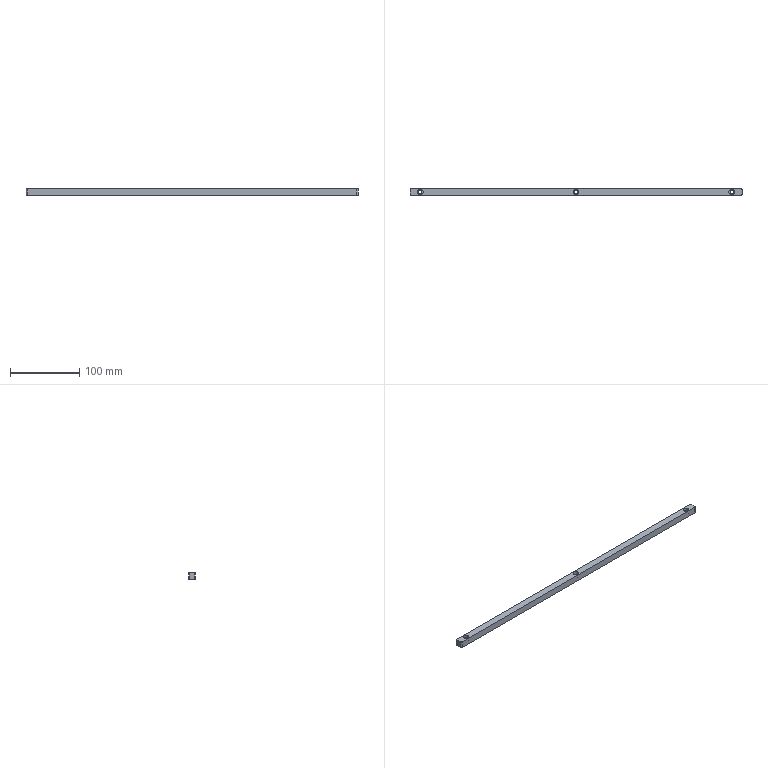Component | SolidWorks | SL010-LeftStreamline-1-1_SL010-02047843SupportBar1-1-1 | 1 solid | 25 faces | box 480 x 10 x 10 mm | volume 47035 mm3 | cylinder 16 | plane 9 | commonest cylinder face diameters 8 x6 4.5 x6 4 x4 | material White POM
STEP:
#1=CARTESIAN_POINT('',(18.937,-4.583,-25.096));
#2=VERTEX_POINT('',#1);
#3=CARTESIAN_POINT('',(19.252,-4.583,-25.096));
#4=VERTEX_POINT('',#3);
#5=CARTESIAN_POINT('',(19.094,-4.583,-25.096));
#6=DIRECTION('',(0.,0.,1.));
#7=DIRECTION('',(1.,0.,0.));
#8=AXIS2_PLACEMENT_3D('',#5,#6,#7);
#9=CIRCLE('',#8,0.1575);
#10=EDGE_CURVE('',#2,#4,#9,.T.);
#11=ORIENTED_EDGE('',*,*,#10,.F.);
#12=CARTESIAN_POINT('',(18.937,-4.583,-24.923));
#13=VERTEX_POINT('',#12);
#14=CARTESIAN_POINT('',(18.937,-4.583,-24.923));
#15=DIRECTION('',(0.,0.,1.));
#16=VECTOR('',#15,39.37);
#17=LINE('',#14,#16);
#18=EDGE_CURVE('',#2,#13,#17,.T.);
#19=ORIENTED_EDGE('',*,*,#18,.T.);
#20=CARTESIAN_POINT('',(19.252,-4.583,-24.923));
#21=VERTEX_POINT('',#20);
#22=CARTESIAN_POINT('',(19.094,-4.583,-24.923));
#23=DIRECTION('',(0.,0.,1.));
#24=DIRECTION('',(1.,0.,0.));
#25=AXIS2_PLACEMENT_3D('',#22,#23,#24);
#26=CIRCLE('',#25,0.1575);
#27=EDGE_CURVE('',#13,#21,#26,.T.);
#28=ORIENTED_EDGE('',*,*,#27,.T.);
#29=CARTESIAN_POINT('',(19.252,-4.583,-24.923));
#30=DIRECTION('',(0.,0.,1.));
#31=VECTOR('',#30,39.37);
#32=LINE('',#29,#31);
#33=EDGE_CURVE('',#4,#21,#32,.T.);
#34=ORIENTED_EDGE('',*,*,#33,.F.);
#35=EDGE_LOOP('',(#11,#19,#28,#34));
#36=FACE_OUTER_BOUND('',#35,.T.);
#37=CARTESIAN_POINT('',(19.094,-4.583,-24.923));
#38=DIRECTION('',(0.,0.,1.));
#39=DIRECTION('',(1.,0.,0.));
#40=AXIS2_PLACEMENT_3D('',#37,#38,#39);
#41=CYLINDRICAL_SURFACE('',#40,0.1575);
#42=ADVANCED_FACE('',(#36),#41,.F.);
#43=CARTESIAN_POINT('',(19.006,-4.583,-25.316));
#44=VERTEX_POINT('',#43);
#45=CARTESIAN_POINT('',(19.183,-4.583,-25.316));
#46=VERTEX_POINT('',#45);
#47=CARTESIAN_POINT('',(19.094,-4.583,-25.316));
#48=DIRECTION('',(0.,0.,1.));
#49=DIRECTION('',(1.,0.,0.));
#50=AXIS2_PLACEMENT_3D('',#47,#48,#49);
#51=CIRCLE('',#50,0.08858);
#52=EDGE_CURVE('',#44,#46,#51,.T.);
#53=ORIENTED_EDGE('',*,*,#52,.F.);
#54=CARTESIAN_POINT('',(19.006,-4.583,-25.096));
#55=VERTEX_POINT('',#54);
#56=CARTESIAN_POINT('',(19.006,-4.583,-24.923));
#57=DIRECTION('',(0.,0.,1.));
#58=VECTOR('',#57,39.37);
#59=LINE('',#56,#58);
#60=EDGE_CURVE('',#44,#55,#59,.T.);
#61=ORIENTED_EDGE('',*,*,#60,.T.);
#62=CARTESIAN_POINT('',(19.183,-4.583,-25.096));
#63=VERTEX_POINT('',#62);
#64=CARTESIAN_POINT('',(19.094,-4.583,-25.096));
#65=DIRECTION('',(0.,0.,1.));
#66=DIRECTION('',(1.,0.,0.));
#67=AXIS2_PLACEMENT_3D('',#64,#65,#66);
#68=CIRCLE('',#67,0.08858);
#69=EDGE_CURVE('',#55,#63,#68,.T.);
#70=ORIENTED_EDGE('',*,*,#69,.T.);
#71=CARTESIAN_POINT('',(19.183,-4.583,-24.923));
#72=DIRECTION('',(0.,0.,1.));
#73=VECTOR('',#72,39.37);
#74=LINE('',#71,#73);
#75=EDGE_CURVE('',#46,#63,#74,.T.);
#76=ORIENTED_EDGE('',*,*,#75,.F.);
#77=EDGE_LOOP('',(#53,#61,#70,#76));
#78=FACE_OUTER_BOUND('',#77,.T.);
#79=CARTESIAN_POINT('',(19.094,-4.583,-24.923));
#80=DIRECTION('',(0.,0.,1.));
#81=DIRECTION('',(1.,0.,0.));
#82=AXIS2_PLACEMENT_3D('',#79,#80,#81);
#83=CYLINDRICAL_SURFACE('',#82,0.08858);
#84=ADVANCED_FACE('',(#78),#83,.F.);
#85=CARTESIAN_POINT('',(36.654,-4.583,-25.096));
#86=VERTEX_POINT('',#85);
#87=CARTESIAN_POINT('',(36.969,-4.583,-25.096));
#88=VERTEX_POINT('',#87);
#89=CARTESIAN_POINT('',(36.811,-4.583,-25.096));
#90=DIRECTION('',(0.,0.,1.));
#91=DIRECTION('',(1.,0.,0.));
#92=AXIS2_PLACEMENT_3D('',#89,#90,#91);
#93=CIRCLE('',#92,0.1575);
#94=EDGE_CURVE('',#86,#88,#93,.T.);
#95=ORIENTED_EDGE('',*,*,#94,.F.);
#96=CARTESIAN_POINT('',(36.654,-4.583,-24.923));
#97=VERTEX_POINT('',#96);
#98=CARTESIAN_POINT('',(36.654,-4.583,-24.923));
#99=DIRECTION('',(0.,0.,1.));
#100=VECTOR('',#99,39.37);
#101=LINE('',#98,#100);
#102=EDGE_CURVE('',#86,#97,#101,.T.);
#103=ORIENTED_EDGE('',*,*,#102,.T.);
#104=CARTESIAN_POINT('',(36.969,-4.583,-24.923));
#105=VERTEX_POINT('',#104);
#106=CARTESIAN_POINT('',(36.811,-4.583,-24.923));
#107=DIRECTION('',(0.,0.,1.));
#108=DIRECTION('',(1.,0.,0.));
#109=AXIS2_PLACEMENT_3D('',#106,#107,#108);
#110=CIRCLE('',#109,0.1575);
#111=EDGE_CURVE('',#97,#105,#110,.T.);
#112=ORIENTED_EDGE('',*,*,#111,.T.);
#113=CARTESIAN_POINT('',(36.969,-4.583,-24.923));
#114=DIRECTION('',(0.,0.,1.));
#115=VECTOR('',#114,39.37);
#116=LINE('',#113,#115);
#117=EDGE_CURVE('',#88,#105,#116,.T.);
#118=ORIENTED_EDGE('',*,*,#117,.F.);
#119=EDGE_LOOP('',(#95,#103,#112,#118));
#120=FACE_OUTER_BOUND('',#119,.T.);
#121=CARTESIAN_POINT('',(36.811,-4.583,-24.923));
#122=DIRECTION('',(0.,0.,1.));
#123=DIRECTION('',(1.,0.,0.));
#124=AXIS2_PLACEMENT_3D('',#121,#122,#123);
#125=CYLINDRICAL_SURFACE('',#124,0.1575);
#126=ADVANCED_FACE('',(#120),#125,.F.);
#127=CARTESIAN_POINT('',(36.722,-4.583,-25.316));
#128=VERTEX_POINT('',#127);
#129=CARTESIAN_POINT('',(36.9,-4.583,-25.316));
#130=VERTEX_POINT('',#129);
#131=CARTESIAN_POINT('',(36.811,-4.583,-25.316));
#132=DIRECTION('',(0.,0.,1.));
#133=DIRECTION('',(1.,0.,0.));
#134=AXIS2_PLACEMENT_3D('',#131,#132,#133);
#135=CIRCLE('',#134,0.08858);
#136=EDGE_CURVE('',#128,#130,#135,.T.);
#137=ORIENTED_EDGE('',*,*,#136,.F.);
#138=CARTESIAN_POINT('',(36.722,-4.583,-25.096));
#139=VERTEX_POINT('',#138);
#140=CARTESIAN_POINT('',(36.722,-4.583,-24.923));
#141=DIRECTION('',(0.,0.,1.));
#142=VECTOR('',#141,39.37);
#143=LINE('',#140,#142);
#144=EDGE_CURVE('',#128,#139,#143,.T.);
#145=ORIENTED_EDGE('',*,*,#144,.T.);
#146=CARTESIAN_POINT('',(36.9,-4.583,-25.096));
#147=VERTEX_POINT('',#146);
#148=CARTESIAN_POINT('',(36.811,-4.583,-25.096));
#149=DIRECTION('',(0.,0.,1.));
#150=DIRECTION('',(1.,0.,0.));
#151=AXIS2_PLACEMENT_3D('',#148,#149,#150);
#152=CIRCLE('',#151,0.08858);
#153=EDGE_CURVE('',#139,#147,#152,.T.);
#154=ORIENTED_EDGE('',*,*,#153,.T.);
#155=CARTESIAN_POINT('',(36.9,-4.583,-24.923));
#156=DIRECTION('',(0.,0.,1.));
#157=VECTOR('',#156,39.37);
#158=LINE('',#155,#157);
#159=EDGE_CURVE('',#130,#147,#158,.T.);
#160=ORIENTED_EDGE('',*,*,#159,.F.);
#161=EDGE_LOOP('',(#137,#145,#154,#160));
#162=FACE_OUTER_BOUND('',#161,.T.);
#163=CARTESIAN_POINT('',(36.811,-4.583,-24.923));
#164=DIRECTION('',(0.,0.,1.));
#165=DIRECTION('',(1.,0.,0.));
#166=AXIS2_PLACEMENT_3D('',#163,#164,#165);
#167=CYLINDRICAL_SURFACE('',#166,0.08858);
#168=ADVANCED_FACE('',(#162),#167,.F.);
#169=CARTESIAN_POINT('',(27.795,-4.583,-25.096));
#170=VERTEX_POINT('',#169);
#171=CARTESIAN_POINT('',(28.11,-4.583,-25.096));
#172=VERTEX_POINT('',#171);
#173=CARTESIAN_POINT('',(27.953,-4.583,-25.096));
#174=DIRECTION('',(0.,0.,1.));
#175=DIRECTION('',(1.,0.,0.));
#176=AXIS2_PLACEMENT_3D('',#173,#174,#175);
#177=CIRCLE('',#176,0.1575);
#178=EDGE_CURVE('',#170,#172,#177,.T.);
#179=ORIENTED_EDGE('',*,*,#178,.F.);
#180=CARTESIAN_POINT('',(27.795,-4.583,-24.923));
#181=VERTEX_POINT('',#180);
#182=CARTESIAN_POINT('',(27.795,-4.583,-24.923));
#183=DIRECTION('',(0.,0.,1.));
#184=VECTOR('',#183,39.37);
#185=LINE('',#182,#184);
#186=EDGE_CURVE('',#170,#181,#185,.T.);
#187=ORIENTED_EDGE('',*,*,#186,.T.);
#188=CARTESIAN_POINT('',(28.11,-4.583,-24.923));
#189=VERTEX_POINT('',#188);
#190=CARTESIAN_POINT('',(27.953,-4.583,-24.923));
#191=DIRECTION('',(0.,0.,1.));
#192=DIRECTION('',(1.,0.,0.));
#193=AXIS2_PLACEMENT_3D('',#190,#191,#192);
#194=CIRCLE('',#193,0.1575);
#195=EDGE_CURVE('',#181,#189,#194,.T.);
#196=ORIENTED_EDGE('',*,*,#195,.T.);
#197=CARTESIAN_POINT('',(28.11,-4.583,-24.923));
#198=DIRECTION('',(0.,0.,1.));
#199=VECTOR('',#198,39.37);
#200=LINE('',#197,#199);
#201=EDGE_CURVE('',#172,#189,#200,.T.);
#202=ORIENTED_EDGE('',*,*,#201,.F.);
#203=EDGE_LOOP('',(#179,#187,#196,#202));
#204=FACE_OUTER_BOUND('',#203,.T.);
#205=CARTESIAN_POINT('',(27.953,-4.583,-24.923));
#206=DIRECTION('',(0.,0.,1.));
#207=DIRECTION('',(1.,0.,0.));
#208=AXIS2_PLACEMENT_3D('',#205,#206,#207);
#209=CYLINDRICAL_SURFACE('',#208,0.1575);
#210=ADVANCED_FACE('',(#204),#209,.F.);
#211=CARTESIAN_POINT('',(27.864,-4.583,-25.316));
#212=VERTEX_POINT('',#211);
#213=CARTESIAN_POINT('',(28.041,-4.583,-25.316));
#214=VERTEX_POINT('',#213);
#215=CARTESIAN_POINT('',(27.953,-4.583,-25.316));
#216=DIRECTION('',(0.,0.,1.));
#217=DIRECTION('',(1.,0.,0.));
#218=AXIS2_PLACEMENT_3D('',#215,#216,#217);
#219=CIRCLE('',#218,0.08858);
#220=EDGE_CURVE('',#212,#214,#219,.T.);
#221=ORIENTED_EDGE('',*,*,#220,.F.);
#222=CARTESIAN_POINT('',(27.864,-4.583,-25.096));
#223=VERTEX_POINT('',#222);
#224=CARTESIAN_POINT('',(27.864,-4.583,-24.923));
#225=DIRECTION('',(0.,0.,1.));
#226=VECTOR('',#225,39.37);
#227=LINE('',#224,#226);
#228=EDGE_CURVE('',#212,#223,#227,.T.);
#229=ORIENTED_EDGE('',*,*,#228,.T.);
#230=CARTESIAN_POINT('',(28.041,-4.583,-25.096));
#231=VERTEX_POINT('',#230);
#232=CARTESIAN_POINT('',(27.953,-4.583,-25.096));
#233=DIRECTION('',(0.,0.,1.));
#234=DIRECTION('',(1.,0.,0.));
#235=AXIS2_PLACEMENT_3D('',#232,#233,#234);
#236=CIRCLE('',#235,0.08858);
#237=EDGE_CURVE('',#223,#231,#236,.T.);
#238=ORIENTED_EDGE('',*,*,#237,.T.);
#239=CARTESIAN_POINT('',(28.041,-4.583,-24.923));
#240=DIRECTION('',(0.,0.,1.));
#241=VECTOR('',#240,39.37);
#242=LINE('',#239,#241);
#243=EDGE_CURVE('',#214,#231,#242,.T.);
#244=ORIENTED_EDGE('',*,*,#243,.F.);
#245=EDGE_LOOP('',(#221,#229,#238,#244));
#246=FACE_OUTER_BOUND('',#245,.T.);
#247=CARTESIAN_POINT('',(27.953,-4.583,-24.923));
#248=DIRECTION('',(0.,0.,1.));
#249=DIRECTION('',(1.,0.,0.));
#250=AXIS2_PLACEMENT_3D('',#247,#248,#249);
#251=CYLINDRICAL_SURFACE('',#250,0.08858);
#252=ADVANCED_FACE('',(#246),#251,.F.);
#253=CARTESIAN_POINT('',(37.402,-4.701,-24.923));
#254=VERTEX_POINT('',#253);
#255=CARTESIAN_POINT('',(37.402,-4.465,-24.923));
#256=VERTEX_POINT('',#255);
#257=CARTESIAN_POINT('',(37.402,-4.386,-24.923));
#258=DIRECTION('',(0.,1.,0.));
#259=VECTOR('',#258,39.37);
#260=LINE('',#257,#259);
#261=EDGE_CURVE('',#254,#256,#260,.T.);
#262=ORIENTED_EDGE('',*,*,#261,.F.);
#263=CARTESIAN_POINT('',(37.402,-4.701,-25.316));
#264=VERTEX_POINT('',#263);
#265=CARTESIAN_POINT('',(37.402,-4.701,-24.923));
#266=DIRECTION('',(0.,0.,-1.));
#267=VECTOR('',#266,39.37);
#268=LINE('',#265,#267);
#269=EDGE_CURVE('',#254,#264,#268,.T.);
#270=ORIENTED_EDGE('',*,*,#269,.T.);
#271=CARTESIAN_POINT('',(37.402,-4.465,-25.316));
#272=VERTEX_POINT('',#271);
#273=CARTESIAN_POINT('',(37.402,-4.386,-25.316));
#274=DIRECTION('',(0.,1.,0.));
#275=VECTOR('',#274,39.37);
#276=LINE('',#273,#275);
#277=EDGE_CURVE('',#264,#272,#276,.T.);
#278=ORIENTED_EDGE('',*,*,#277,.T.);
#279=CARTESIAN_POINT('',(37.402,-4.465,-24.923));
#280=DIRECTION('',(0.,0.,1.));
#281=VECTOR('',#280,39.37);
#282=LINE('',#279,#281);
#283=EDGE_CURVE('',#272,#256,#282,.T.);
#284=ORIENTED_EDGE('',*,*,#283,.T.);
#285=EDGE_LOOP('',(#262,#270,#278,#284));
#286=FACE_OUTER_BOUND('',#285,.T.);
#287=CARTESIAN_POINT('',(37.402,-4.386,-24.923));
#288=DIRECTION('',(-1.,0.,0.));
#289=DIRECTION('',(0.,0.,1.));
#290=AXIS2_PLACEMENT_3D('',#287,#288,#289);
#291=PLANE('',#290);
#292=ADVANCED_FACE('',(#286),#291,.F.);
#293=CARTESIAN_POINT('',(37.323,-4.386,-24.923));
#294=VERTEX_POINT('',#293);
#295=CARTESIAN_POINT('',(18.583,-4.386,-24.923));
#296=VERTEX_POINT('',#295);
#297=CARTESIAN_POINT('',(18.504,-4.386,-24.923));
#298=DIRECTION('',(-1.,0.,0.));
#299=VECTOR('',#298,39.37);
#300=LINE('',#297,#299);
#301=EDGE_CURVE('',#294,#296,#300,.T.);
#302=ORIENTED_EDGE('',*,*,#301,.F.);
#303=CARTESIAN_POINT('',(37.323,-4.386,-25.316));
#304=VERTEX_POINT('',#303);
#305=CARTESIAN_POINT('',(37.323,-4.386,-24.923));
#306=DIRECTION('',(0.,0.,-1.));
#307=VECTOR('',#306,39.37);
#308=LINE('',#305,#307);
#309=EDGE_CURVE('',#294,#304,#308,.T.);
#310=ORIENTED_EDGE('',*,*,#309,.T.);
#311=CARTESIAN_POINT('',(18.583,-4.386,-25.316));
#312=VERTEX_POINT('',#311);
#313=CARTESIAN_POINT('',(18.504,-4.386,-25.316));
#314=DIRECTION('',(-1.,0.,0.));
#315=VECTOR('',#314,39.37);
#316=LINE('',#313,#315);
#317=EDGE_CURVE('',#304,#312,#316,.T.);
#318=ORIENTED_EDGE('',*,*,#317,.T.);
#319=CARTESIAN_POINT('',(18.583,-4.386,-24.923));
#320=DIRECTION('',(0.,0.,1.));
#321=VECTOR('',#320,39.37);
#322=LINE('',#319,#321);
#323=EDGE_CURVE('',#312,#296,#322,.T.);
#324=ORIENTED_EDGE('',*,*,#323,.T.);
#325=EDGE_LOOP('',(#302,#310,#318,#324));
#326=FACE_OUTER_BOUND('',#325,.T.);
#327=CARTESIAN_POINT('',(18.504,-4.386,-24.923));
#328=DIRECTION('',(0.,-1.,0.));
#329=DIRECTION('',(0.,0.,-1.));
#330=AXIS2_PLACEMENT_3D('',#327,#328,#329);
#331=PLANE('',#330);
#332=ADVANCED_FACE('',(#326),#331,.F.);
#333=CARTESIAN_POINT('',(18.504,-4.465,-25.316));
#334=VERTEX_POINT('',#333);
#335=CARTESIAN_POINT('',(18.504,-4.701,-25.316));
#336=VERTEX_POINT('',#335);
#337=CARTESIAN_POINT('',(18.504,-4.386,-25.316));
#338=DIRECTION('',(0.,-1.,0.));
#339=VECTOR('',#338,39.37);
#340=LINE('',#337,#339);
#341=EDGE_CURVE('',#334,#336,#340,.T.);
#342=ORIENTED_EDGE('',*,*,#341,.T.);
#343=CARTESIAN_POINT('',(18.504,-4.701,-24.923));
#344=VERTEX_POINT('',#343);
#345=CARTESIAN_POINT('',(18.504,-4.701,-24.923));
#346=DIRECTION('',(0.,0.,1.));
#347=VECTOR('',#346,39.37);
#348=LINE('',#345,#347);
#349=EDGE_CURVE('',#336,#344,#348,.T.);
#350=ORIENTED_EDGE('',*,*,#349,.T.);
#351=CARTESIAN_POINT('',(18.504,-4.465,-24.923));
#352=VERTEX_POINT('',#351);
#353=CARTESIAN_POINT('',(18.504,-4.386,-24.923));
#354=DIRECTION('',(0.,-1.,0.));
#355=VECTOR('',#354,39.37);
#356=LINE('',#353,#355);
#357=EDGE_CURVE('',#352,#344,#356,.T.);
#358=ORIENTED_EDGE('',*,*,#357,.F.);
#359=CARTESIAN_POINT('',(18.504,-4.465,-24.923));
#360=DIRECTION('',(0.,0.,-1.));
#361=VECTOR('',#360,39.37);
#362=LINE('',#359,#361);
#363=EDGE_CURVE('',#352,#334,#362,.T.);
#364=ORIENTED_EDGE('',*,*,#363,.T.);
#365=EDGE_LOOP('',(#342,#350,#358,#364));
#366=FACE_OUTER_BOUND('',#365,.T.);
#367=CARTESIAN_POINT('',(18.504,-4.386,-24.923));
#368=DIRECTION('',(1.,0.,0.));
#369=DIRECTION('',(0.,0.,-1.));
#370=AXIS2_PLACEMENT_3D('',#367,#368,#369);
#371=PLANE('',#370);
#372=ADVANCED_FACE('',(#366),#371,.F.);
#373=CARTESIAN_POINT('',(18.583,-4.78,-25.316));
#374=VERTEX_POINT('',#373);
#375=CARTESIAN_POINT('',(37.323,-4.78,-25.316));
#376=VERTEX_POINT('',#375);
#377=CARTESIAN_POINT('',(18.504,-4.78,-25.316));
#378=DIRECTION('',(1.,0.,0.));
#379=VECTOR('',#378,39.37);
#380=LINE('',#377,#379);
#381=EDGE_CURVE('',#374,#376,#380,.T.);
#382=ORIENTED_EDGE('',*,*,#381,.T.);
#383=CARTESIAN_POINT('',(37.323,-4.78,-24.923));
#384=VERTEX_POINT('',#383);
#385=CARTESIAN_POINT('',(37.323,-4.78,-24.923));
#386=DIRECTION('',(0.,0.,1.));
#387=VECTOR('',#386,39.37);
#388=LINE('',#385,#387);
#389=EDGE_CURVE('',#376,#384,#388,.T.);
#390=ORIENTED_EDGE('',*,*,#389,.T.);
#391=CARTESIAN_POINT('',(18.583,-4.78,-24.923));
#392=VERTEX_POINT('',#391);
#393=CARTESIAN_POINT('',(18.504,-4.78,-24.923));
#394=DIRECTION('',(1.,0.,0.));
#395=VECTOR('',#394,39.37);
#396=LINE('',#393,#395);
#397=EDGE_CURVE('',#392,#384,#396,.T.);
#398=ORIENTED_EDGE('',*,*,#397,.F.);
#399=CARTESIAN_POINT('',(18.583,-4.78,-24.923));
#400=DIRECTION('',(0.,0.,-1.));
#401=VECTOR('',#400,39.37);
#402=LINE('',#399,#401);
#403=EDGE_CURVE('',#392,#374,#402,.T.);
#404=ORIENTED_EDGE('',*,*,#403,.T.);
#405=EDGE_LOOP('',(#382,#390,#398,#404));
#406=FACE_OUTER_BOUND('',#405,.T.);
#407=CARTESIAN_POINT('',(18.504,-4.78,-24.923));
#408=DIRECTION('',(0.,1.,0.));
#409=DIRECTION('',(0.,0.,1.));
#410=AXIS2_PLACEMENT_3D('',#407,#408,#409);
#411=PLANE('',#410);
#412=ADVANCED_FACE('',(#406),#411,.F.);
#413=CARTESIAN_POINT('',(19.094,-4.583,-24.923));
#414=DIRECTION('',(0.,0.,1.));
#415=DIRECTION('',(1.,0.,0.));
#416=AXIS2_PLACEMENT_3D('',#413,#414,#415);
#417=CIRCLE('',#416,0.1575);
#418=EDGE_CURVE('',#21,#13,#417,.T.);
#419=ORIENTED_EDGE('',*,*,#418,.F.);
#420=ORIENTED_EDGE('',*,*,#27,.F.);
#421=EDGE_LOOP('',(#419,#420));
#422=FACE_BOUND('',#421,.T.);
#423=CARTESIAN_POINT('',(36.811,-4.583,-24.923));
#424=DIRECTION('',(0.,0.,1.));
#425=DIRECTION('',(1.,0.,0.));
#426=AXIS2_PLACEMENT_3D('',#423,#424,#425);
#427=CIRCLE('',#426,0.1575);
#428=EDGE_CURVE('',#105,#97,#427,.T.);
#429=ORIENTED_EDGE('',*,*,#428,.F.);
#430=ORIENTED_EDGE('',*,*,#111,.F.);
#431=EDGE_LOOP('',(#429,#430));
#432=FACE_BOUND('',#431,.T.);
#433=CARTESIAN_POINT('',(27.953,-4.583,-24.923));
#434=DIRECTION('',(0.,0.,1.));
#435=DIRECTION('',(1.,0.,0.));
#436=AXIS2_PLACEMENT_3D('',#433,#434,#435);
#437=CIRCLE('',#436,0.1575);
#438=EDGE_CURVE('',#189,#181,#437,.T.);
#439=ORIENTED_EDGE('',*,*,#438,.F.);
#440=ORIENTED_EDGE('',*,*,#195,.F.);
#441=EDGE_LOOP('',(#439,#440));
#442=FACE_BOUND('',#441,.T.);
#443=ORIENTED_EDGE('',*,*,#397,.T.);
#444=CARTESIAN_POINT('',(37.323,-4.701,-24.923));
#445=DIRECTION('',(0.,0.,1.));
#446=DIRECTION('',(1.,0.,0.));
#447=AXIS2_PLACEMENT_3D('',#444,#445,#446);
#448=CIRCLE('',#447,0.07874);
#449=EDGE_CURVE('',#384,#254,#448,.T.);
#450=ORIENTED_EDGE('',*,*,#449,.T.);
#451=ORIENTED_EDGE('',*,*,#261,.T.);
#452=CARTESIAN_POINT('',(37.323,-4.465,-24.923));
#453=DIRECTION('',(0.,0.,1.));
#454=DIRECTION('',(1.,0.,0.));
#455=AXIS2_PLACEMENT_3D('',#452,#453,#454);
#456=CIRCLE('',#455,0.07874);
#457=EDGE_CURVE('',#256,#294,#456,.T.);
#458=ORIENTED_EDGE('',*,*,#457,.T.);
#459=ORIENTED_EDGE('',*,*,#301,.T.);
#460=CARTESIAN_POINT('',(18.583,-4.465,-24.923));
#461=DIRECTION('',(0.,0.,1.));
#462=DIRECTION('',(1.,0.,0.));
#463=AXIS2_PLACEMENT_3D('',#460,#461,#462);
#464=CIRCLE('',#463,0.07874);
#465=EDGE_CURVE('',#296,#352,#464,.T.);
#466=ORIENTED_EDGE('',*,*,#465,.T.);
#467=ORIENTED_EDGE('',*,*,#357,.T.);
#468=CARTESIAN_POINT('',(18.583,-4.701,-24.923));
#469=DIRECTION('',(0.,0.,1.));
#470=DIRECTION('',(1.,0.,0.));
#471=AXIS2_PLACEMENT_3D('',#468,#469,#470);
#472=CIRCLE('',#471,0.07874);
#473=EDGE_CURVE('',#344,#392,#472,.T.);
#474=ORIENTED_EDGE('',*,*,#473,.T.);
#475=EDGE_LOOP('',(#443,#450,#451,#458,#459,#466,#467,#474));
#476=FACE_OUTER_BOUND('',#475,.T.);
#477=CARTESIAN_POINT('',(27.953,-4.583,-24.923));
#478=DIRECTION('',(0.,0.,1.));
#479=DIRECTION('',(1.,0.,0.));
#480=AXIS2_PLACEMENT_3D('',#477,#478,#479);
#481=PLANE('',#480);
#482=ADVANCED_FACE('',(#422,#432,#442,#476),#481,.T.);
#483=CARTESIAN_POINT('',(19.094,-4.583,-25.316));
#484=DIRECTION('',(0.,0.,1.));
#485=DIRECTION('',(1.,0.,0.));
#486=AXIS2_PLACEMENT_3D('',#483,#484,#485);
#487=CIRCLE('',#486,0.08858);
#488=EDGE_CURVE('',#46,#44,#487,.T.);
#489=ORIENTED_EDGE('',*,*,#488,.T.);
#490=ORIENTED_EDGE('',*,*,#52,.T.);
#491=EDGE_LOOP('',(#489,#490));
#492=FACE_BOUND('',#491,.T.);
#493=CARTESIAN_POINT('',(36.811,-4.583,-25.316));
#494=DIRECTION('',(0.,0.,1.));
#495=DIRECTION('',(1.,0.,0.));
#496=AXIS2_PLACEMENT_3D('',#493,#494,#495);
#497=CIRCLE('',#496,0.08858);
#498=EDGE_CURVE('',#130,#128,#497,.T.);
#499=ORIENTED_EDGE('',*,*,#498,.T.);
#500=ORIENTED_EDGE('',*,*,#136,.T.);
#501=EDGE_LOOP('',(#499,#500));
#502=FACE_BOUND('',#501,.T.);
#503=CARTESIAN_POINT('',(27.953,-4.583,-25.316));
#504=DIRECTION('',(0.,0.,1.));
#505=DIRECTION('',(1.,0.,0.));
#506=AXIS2_PLACEMENT_3D('',#503,#504,#505);
#507=CIRCLE('',#506,0.08858);
#508=EDGE_CURVE('',#214,#212,#507,.T.);
#509=ORIENTED_EDGE('',*,*,#508,.T.);
#510=ORIENTED_EDGE('',*,*,#220,.T.);
#511=EDGE_LOOP('',(#509,#510));
#512=FACE_BOUND('',#511,.T.);
#513=ORIENTED_EDGE('',*,*,#277,.F.);
#514=CARTESIAN_POINT('',(37.323,-4.701,-25.316));
#515=DIRECTION('',(0.,0.,-1.));
#516=DIRECTION('',(1.,0.,0.));
#517=AXIS2_PLACEMENT_3D('',#514,#515,#516);
#518=CIRCLE('',#517,0.07874);
#519=EDGE_CURVE('',#264,#376,#518,.T.);
#520=ORIENTED_EDGE('',*,*,#519,.T.);
#521=ORIENTED_EDGE('',*,*,#381,.F.);
#522=CARTESIAN_POINT('',(18.583,-4.701,-25.316));
#523=DIRECTION('',(0.,0.,-1.));
#524=DIRECTION('',(1.,0.,0.));
#525=AXIS2_PLACEMENT_3D('',#522,#523,#524);
#526=CIRCLE('',#525,0.07874);
#527=EDGE_CURVE('',#374,#336,#526,.T.);
#528=ORIENTED_EDGE('',*,*,#527,.T.);
#529=ORIENTED_EDGE('',*,*,#341,.F.);
#530=CARTESIAN_POINT('',(18.583,-4.465,-25.316));
#531=DIRECTION('',(0.,0.,-1.));
#532=DIRECTION('',(1.,0.,0.));
#533=AXIS2_PLACEMENT_3D('',#530,#531,#532);
#534=CIRCLE('',#533,0.07874);
#535=EDGE_CURVE('',#334,#312,#534,.T.);
#536=ORIENTED_EDGE('',*,*,#535,.T.);
#537=ORIENTED_EDGE('',*,*,#317,.F.);
#538=CARTESIAN_POINT('',(37.323,-4.465,-25.316));
#539=DIRECTION('',(0.,0.,-1.));
#540=DIRECTION('',(1.,0.,0.));
#541=AXIS2_PLACEMENT_3D('',#538,#539,#540);
#542=CIRCLE('',#541,0.07874);
#543=EDGE_CURVE('',#304,#272,#542,.T.);
#544=ORIENTED_EDGE('',*,*,#543,.T.);
#545=EDGE_LOOP('',(#513,#520,#521,#528,#529,#536,#537,#544));
#546=FACE_OUTER_BOUND('',#545,.T.);
#547=CARTESIAN_POINT('',(27.953,-4.583,-25.316));
#548=DIRECTION('',(0.,0.,1.));
#549=DIRECTION('',(1.,0.,0.));
#550=AXIS2_PLACEMENT_3D('',#547,#548,#549);
#551=PLANE('',#550);
#552=ADVANCED_FACE('',(#492,#502,#512,#546),#551,.F.);
#553=ORIENTED_EDGE('',*,*,#228,.F.);
#554=ORIENTED_EDGE('',*,*,#508,.F.);
#555=ORIENTED_EDGE('',*,*,#243,.T.);
#556=CARTESIAN_POINT('',(27.953,-4.583,-25.096));
#557=DIRECTION('',(0.,0.,1.));
#558=DIRECTION('',(1.,0.,0.));
#559=AXIS2_PLACEMENT_3D('',#556,#557,#558);
#560=CIRCLE('',#559,0.08858);
#561=EDGE_CURVE('',#231,#223,#560,.T.);
#562=ORIENTED_EDGE('',*,*,#561,.T.);
#563=EDGE_LOOP('',(#553,#554,#555,#562));
#564=FACE_OUTER_BOUND('',#563,.T.);
#565=CARTESIAN_POINT('',(27.953,-4.583,-24.923));
#566=DIRECTION('',(0.,0.,1.));
#567=DIRECTION('',(1.,0.,0.));
#568=AXIS2_PLACEMENT_3D('',#565,#566,#567);
#569=CYLINDRICAL_SURFACE('',#568,0.08858);
#570=ADVANCED_FACE('',(#564),#569,.F.);
#571=ORIENTED_EDGE('',*,*,#561,.F.);
#572=ORIENTED_EDGE('',*,*,#237,.F.);
#573=EDGE_LOOP('',(#571,#572));
#574=FACE_BOUND('',#573,.T.);
#575=CARTESIAN_POINT('',(27.953,-4.583,-25.096));
#576=DIRECTION('',(0.,0.,1.));
#577=DIRECTION('',(1.,0.,0.));
#578=AXIS2_PLACEMENT_3D('',#575,#576,#577);
#579=CIRCLE('',#578,0.1575);
#580=EDGE_CURVE('',#172,#170,#579,.T.);
#581=ORIENTED_EDGE('',*,*,#580,.T.);
#582=ORIENTED_EDGE('',*,*,#178,.T.);
#583=EDGE_LOOP('',(#581,#582));
#584=FACE_OUTER_BOUND('',#583,.T.);
#585=CARTESIAN_POINT('',(28.041,-4.583,-25.096));
#586=DIRECTION('',(0.,0.,-1.));
#587=DIRECTION('',(-1.,0.,0.));
#588=AXIS2_PLACEMENT_3D('',#585,#586,#587);
#589=PLANE('',#588);
#590=ADVANCED_FACE('',(#574,#584),#589,.F.);
#591=ORIENTED_EDGE('',*,*,#186,.F.);
#592=ORIENTED_EDGE('',*,*,#580,.F.);
#593=ORIENTED_EDGE('',*,*,#201,.T.);
#594=ORIENTED_EDGE('',*,*,#438,.T.);
#595=EDGE_LOOP('',(#591,#592,#593,#594));
#596=FACE_OUTER_BOUND('',#595,.T.);
#597=CARTESIAN_POINT('',(27.953,-4.583,-24.923));
#598=DIRECTION('',(0.,0.,1.));
#599=DIRECTION('',(1.,0.,0.));
#600=AXIS2_PLACEMENT_3D('',#597,#598,#599);
#601=CYLINDRICAL_SURFACE('',#600,0.1575);
#602=ADVANCED_FACE('',(#596),#601,.F.);
#603=ORIENTED_EDGE('',*,*,#144,.F.);
#604=ORIENTED_EDGE('',*,*,#498,.F.);
#605=ORIENTED_EDGE('',*,*,#159,.T.);
#606=CARTESIAN_POINT('',(36.811,-4.583,-25.096));
#607=DIRECTION('',(0.,0.,1.));
#608=DIRECTION('',(1.,0.,0.));
#609=AXIS2_PLACEMENT_3D('',#606,#607,#608);
#610=CIRCLE('',#609,0.08858);
#611=EDGE_CURVE('',#147,#139,#610,.T.);
#612=ORIENTED_EDGE('',*,*,#611,.T.);
#613=EDGE_LOOP('',(#603,#604,#605,#612));
#614=FACE_OUTER_BOUND('',#613,.T.);
#615=CARTESIAN_POINT('',(36.811,-4.583,-24.923));
#616=DIRECTION('',(0.,0.,1.));
#617=DIRECTION('',(1.,0.,0.));
#618=AXIS2_PLACEMENT_3D('',#615,#616,#617);
#619=CYLINDRICAL_SURFACE('',#618,0.08858);
#620=ADVANCED_FACE('',(#614),#619,.F.);
#621=ORIENTED_EDGE('',*,*,#611,.F.);
#622=ORIENTED_EDGE('',*,*,#153,.F.);
#623=EDGE_LOOP('',(#621,#622));
#624=FACE_BOUND('',#623,.T.);
#625=CARTESIAN_POINT('',(36.811,-4.583,-25.096));
#626=DIRECTION('',(0.,0.,1.));
#627=DIRECTION('',(1.,0.,0.));
#628=AXIS2_PLACEMENT_3D('',#625,#626,#627);
#629=CIRCLE('',#628,0.1575);
#630=EDGE_CURVE('',#88,#86,#629,.T.);
#631=ORIENTED_EDGE('',*,*,#630,.T.);
#632=ORIENTED_EDGE('',*,*,#94,.T.);
#633=EDGE_LOOP('',(#631,#632));
#634=FACE_OUTER_BOUND('',#633,.T.);
#635=CARTESIAN_POINT('',(36.9,-4.583,-25.096));
#636=DIRECTION('',(0.,0.,-1.));
#637=DIRECTION('',(-1.,0.,0.));
#638=AXIS2_PLACEMENT_3D('',#635,#636,#637);
#639=PLANE('',#638);
#640=ADVANCED_FACE('',(#624,#634),#639,.F.);
#641=ORIENTED_EDGE('',*,*,#102,.F.);
#642=ORIENTED_EDGE('',*,*,#630,.F.);
#643=ORIENTED_EDGE('',*,*,#117,.T.);
#644=ORIENTED_EDGE('',*,*,#428,.T.);
#645=EDGE_LOOP('',(#641,#642,#643,#644));
#646=FACE_OUTER_BOUND('',#645,.T.);
#647=CARTESIAN_POINT('',(36.811,-4.583,-24.923));
#648=DIRECTION('',(0.,0.,1.));
#649=DIRECTION('',(1.,0.,0.));
#650=AXIS2_PLACEMENT_3D('',#647,#648,#649);
#651=CYLINDRICAL_SURFACE('',#650,0.1575);
#652=ADVANCED_FACE('',(#646),#651,.F.);
#653=ORIENTED_EDGE('',*,*,#60,.F.);
#654=ORIENTED_EDGE('',*,*,#488,.F.);
#655=ORIENTED_EDGE('',*,*,#75,.T.);
#656=CARTESIAN_POINT('',(19.094,-4.583,-25.096));
#657=DIRECTION('',(0.,0.,1.));
#658=DIRECTION('',(1.,0.,0.));
#659=AXIS2_PLACEMENT_3D('',#656,#657,#658);
#660=CIRCLE('',#659,0.08858);
#661=EDGE_CURVE('',#63,#55,#660,.T.);
#662=ORIENTED_EDGE('',*,*,#661,.T.);
#663=EDGE_LOOP('',(#653,#654,#655,#662));
#664=FACE_OUTER_BOUND('',#663,.T.);
#665=CARTESIAN_POINT('',(19.094,-4.583,-24.923));
#666=DIRECTION('',(0.,0.,1.));
#667=DIRECTION('',(1.,0.,0.));
#668=AXIS2_PLACEMENT_3D('',#665,#666,#667);
#669=CYLINDRICAL_SURFACE('',#668,0.08858);
#670=ADVANCED_FACE('',(#664),#669,.F.);
#671=ORIENTED_EDGE('',*,*,#661,.F.);
#672=ORIENTED_EDGE('',*,*,#69,.F.);
#673=EDGE_LOOP('',(#671,#672));
#674=FACE_BOUND('',#673,.T.);
#675=CARTESIAN_POINT('',(19.094,-4.583,-25.096));
#676=DIRECTION('',(0.,0.,1.));
#677=DIRECTION('',(1.,0.,0.));
#678=AXIS2_PLACEMENT_3D('',#675,#676,#677);
#679=CIRCLE('',#678,0.1575);
#680=EDGE_CURVE('',#4,#2,#679,.T.);
#681=ORIENTED_EDGE('',*,*,#680,.T.);
#682=ORIENTED_EDGE('',*,*,#10,.T.);
#683=EDGE_LOOP('',(#681,#682));
#684=FACE_OUTER_BOUND('',#683,.T.);
#685=CARTESIAN_POINT('',(19.183,-4.583,-25.096));
#686=DIRECTION('',(0.,0.,-1.));
#687=DIRECTION('',(-1.,0.,0.));
#688=AXIS2_PLACEMENT_3D('',#685,#686,#687);
#689=PLANE('',#688);
#690=ADVANCED_FACE('',(#674,#684),#689,.F.);
#691=ORIENTED_EDGE('',*,*,#18,.F.);
#692=ORIENTED_EDGE('',*,*,#680,.F.);
#693=ORIENTED_EDGE('',*,*,#33,.T.);
#694=ORIENTED_EDGE('',*,*,#418,.T.);
#695=EDGE_LOOP('',(#691,#692,#693,#694));
#696=FACE_OUTER_BOUND('',#695,.T.);
#697=CARTESIAN_POINT('',(19.094,-4.583,-24.923));
#698=DIRECTION('',(0.,0.,1.));
#699=DIRECTION('',(1.,0.,0.));
#700=AXIS2_PLACEMENT_3D('',#697,#698,#699);
#701=CYLINDRICAL_SURFACE('',#700,0.1575);
#702=ADVANCED_FACE('',(#696),#701,.F.);
#703=ORIENTED_EDGE('',*,*,#449,.F.);
#704=ORIENTED_EDGE('',*,*,#389,.F.);
#705=ORIENTED_EDGE('',*,*,#519,.F.);
#706=ORIENTED_EDGE('',*,*,#269,.F.);
#707=EDGE_LOOP('',(#703,#704,#705,#706));
#708=FACE_OUTER_BOUND('',#707,.T.);
#709=CARTESIAN_POINT('',(37.323,-4.701,-24.923));
#710=DIRECTION('',(0.,0.,-1.));
#711=DIRECTION('',(-1.,0.,0.));
#712=AXIS2_PLACEMENT_3D('',#709,#710,#711);
#713=CYLINDRICAL_SURFACE('',#712,0.07874);
#714=ADVANCED_FACE('',(#708),#713,.T.);
#715=ORIENTED_EDGE('',*,*,#457,.F.);
#716=ORIENTED_EDGE('',*,*,#283,.F.);
#717=ORIENTED_EDGE('',*,*,#543,.F.);
#718=ORIENTED_EDGE('',*,*,#309,.F.);
#719=EDGE_LOOP('',(#715,#716,#717,#718));
#720=FACE_OUTER_BOUND('',#719,.T.);
#721=CARTESIAN_POINT('',(37.323,-4.465,-24.923));
#722=DIRECTION('',(0.,0.,-1.));
#723=DIRECTION('',(-1.,0.,0.));
#724=AXIS2_PLACEMENT_3D('',#721,#722,#723);
#725=CYLINDRICAL_SURFACE('',#724,0.07874);
#726=ADVANCED_FACE('',(#720),#725,.T.);
#727=ORIENTED_EDGE('',*,*,#473,.F.);
#728=ORIENTED_EDGE('',*,*,#349,.F.);
#729=ORIENTED_EDGE('',*,*,#527,.F.);
#730=ORIENTED_EDGE('',*,*,#403,.F.);
#731=EDGE_LOOP('',(#727,#728,#729,#730));
#732=FACE_OUTER_BOUND('',#731,.T.);
#733=CARTESIAN_POINT('',(18.583,-4.701,-24.923));
#734=DIRECTION('',(0.,0.,-1.));
#735=DIRECTION('',(-1.,0.,0.));
#736=AXIS2_PLACEMENT_3D('',#733,#734,#735);
#737=CYLINDRICAL_SURFACE('',#736,0.07874);
#738=ADVANCED_FACE('',(#732),#737,.T.);
#739=ORIENTED_EDGE('',*,*,#465,.F.);
#740=ORIENTED_EDGE('',*,*,#323,.F.);
#741=ORIENTED_EDGE('',*,*,#535,.F.);
#742=ORIENTED_EDGE('',*,*,#363,.F.);
#743=EDGE_LOOP('',(#739,#740,#741,#742));
#744=FACE_OUTER_BOUND('',#743,.T.);
#745=CARTESIAN_POINT('',(18.583,-4.465,-24.923));
#746=DIRECTION('',(0.,0.,-1.));
#747=DIRECTION('',(-1.,0.,0.));
#748=AXIS2_PLACEMENT_3D('',#745,#746,#747);
#749=CYLINDRICAL_SURFACE('',#748,0.07874);
#750=ADVANCED_FACE('',(#744),#749,.T.);
#751=CLOSED_SHELL('',(#42,#84,#126,#168,#210,#252,#292,#332,#372,#412,#482,#552,#570,#590,#602,#620,#640,#652,#670,#690,#702,#714,#726,#738,#750));
#752=MANIFOLD_SOLID_BREP('',#751);
#753=CARTESIAN_POINT('',(0.,0.,0.));
#754=DIRECTION('',(0.,0.,1.));
#755=DIRECTION('',(1.,0.,0.));
#756=AXIS2_PLACEMENT_3D('',#753,#754,#755);
#757=(LENGTH_UNIT()NAMED_UNIT(*)SI_UNIT($,.METRE.));
#758=LENGTH_MEASURE_WITH_UNIT(LENGTH_MEASURE(0.0254),#757);
#759=DIMENSIONAL_EXPONENTS(1.,0.,0.,0.,0.,0.,0.);
#760=(CONVERSION_BASED_UNIT('',#758)LENGTH_UNIT()NAMED_UNIT(#759));
#761=UNCERTAINTY_MEASURE_WITH_UNIT(LENGTH_MEASURE(0.00001),#760,'','');
#762=(NAMED_UNIT(*)PLANE_ANGLE_UNIT()SI_UNIT($,.RADIAN.));
#763=(NAMED_UNIT(*)SI_UNIT($,.STERADIAN.)SOLID_ANGLE_UNIT());
#764=(GEOMETRIC_REPRESENTATION_CONTEXT(3)GLOBAL_UNCERTAINTY_ASSIGNED_CONTEXT((#761))GLOBAL_UNIT_ASSIGNED_CONTEXT((#760,#762,#763))REPRESENTATION_CONTEXT('',''));
#765=ADVANCED_BREP_SHAPE_REPRESENTATION('',(#752,#756),#764);
#766=COLOUR_RGB('',0.7922,0.8196,0.9333);
#767=FILL_AREA_STYLE_COLOUR('',#766);
#768=FILL_AREA_STYLE('',(#767));
#769=SURFACE_STYLE_FILL_AREA(#768);
#770=SURFACE_SIDE_STYLE('',(#769));
#771=SURFACE_STYLE_USAGE(.BOTH.,#770);
#772=PRESENTATION_STYLE_ASSIGNMENT((#771));
#773=STYLED_ITEM('',(#772),#752);
#774=PRESENTATION_LAYER_ASSIGNMENT('','',(#773));
#775=(LENGTH_UNIT()NAMED_UNIT(*)SI_UNIT($,.METRE.));
#776=LENGTH_MEASURE_WITH_UNIT(LENGTH_MEASURE(0.0254),#775);
#777=DIMENSIONAL_EXPONENTS(1.,0.,0.,0.,0.,0.,0.);
#778=(CONVERSION_BASED_UNIT('',#776)LENGTH_UNIT()NAMED_UNIT(#777));
#779=UNCERTAINTY_MEASURE_WITH_UNIT(LENGTH_MEASURE(0.00001),#778,'','');
#780=(NAMED_UNIT(*)PLANE_ANGLE_UNIT()SI_UNIT($,.RADIAN.));
#781=(NAMED_UNIT(*)SI_UNIT($,.STERADIAN.)SOLID_ANGLE_UNIT());
#782=(GEOMETRIC_REPRESENTATION_CONTEXT(3)GLOBAL_UNCERTAINTY_ASSIGNED_CONTEXT((#779))GLOBAL_UNIT_ASSIGNED_CONTEXT((#778,#780,#781))REPRESENTATION_CONTEXT('',''));
#783=MECHANICAL_DESIGN_GEOMETRIC_PRESENTATION_REPRESENTATION('',(#773),#782);